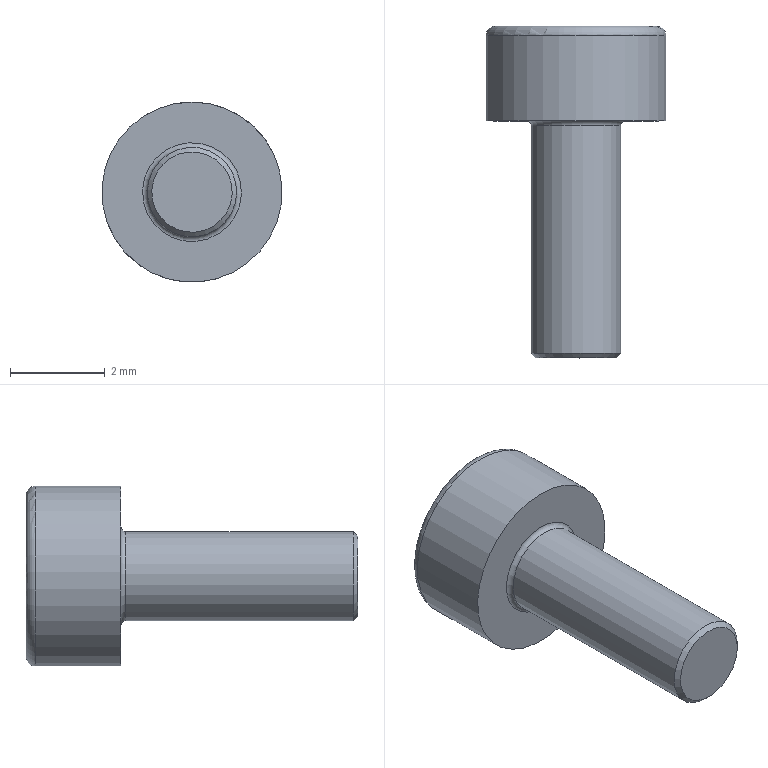Component | NX | GB-T70_1-2000_M2X5 | 1 solid | 27 faces | volume 33 mm3 | plane 15 | cone 8 | cylinder 2 | torus 2 | commonest cylinder face diameters 1.886 x1 3.8 x1